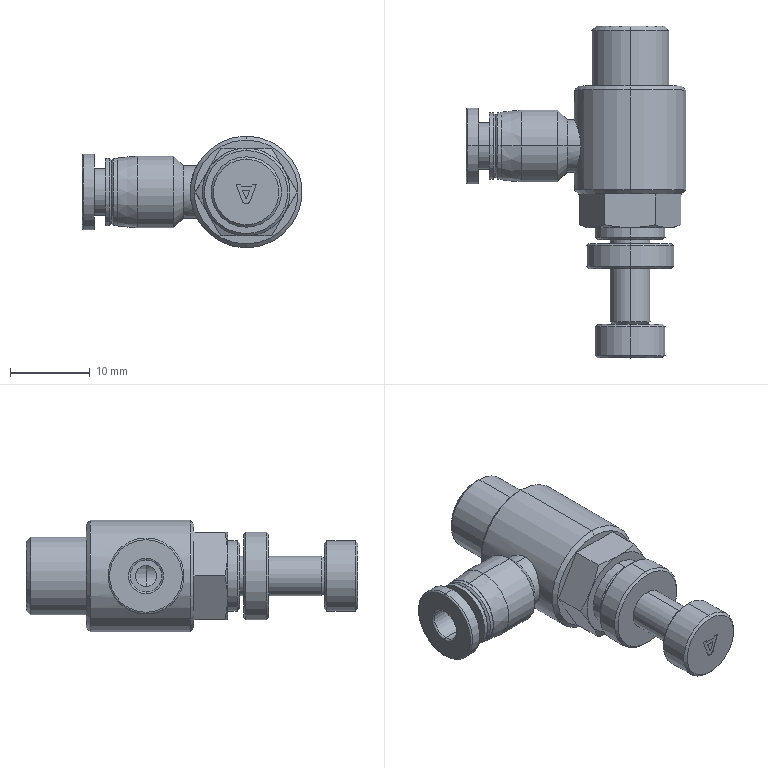Component | SolidWorks | F01AE00111-A2000-21TopEdgeAssembly-1_PSL401A-1 | 1 solid | 109 faces | box 27.5 x 41.5 x 14 mm | volume 4098 mm3 | cylinder 36 | plane 33 | cone 32 | torus 6 | sphere 2 | commonest cylinder face diameters 8.4 x4 8.8 x4 5 x4 2.667 x2 9 x2 5.8 x2 9.5 x2 6.6 x2
build123d program:
from build123d import *

# Parameters (mm, degrees)
SKETCH2_R          = 11
CUT_EXTRUDE1_DEPTH = 4.2
CUT_EXTRUDE2_DEPTH = 0.05


with BuildPart() as part:
    # Sketch1 → Revolve1 (revolve)
    with BuildSketch(Plane.XY, mode=Mode.PRIVATE) as revolve1_sk:
        Polygon((0, -15), (-4.283, -15), (-4.864, -14.419), (-4.864, -7.5), (-6.5, -7.5), (-7, -7), (-7, 5.5), (-6.5, 6), (-6.351, 6), (-6.351, 9.848), (-5.5, 10.2), (-4.4, 10.2), (-4.4, 11.4), (-4.1, 11.7), (-2.5, 11.7), (-2.5, 12.2), (-5.2, 12.2), (-5.5, 12.5), (-5.5, 15.05), (-5.2, 15.35), (-2.5, 15.35), (-2.5, 21.994), (-2.193, 22.3), (-4.1, 22.3), (-4.4, 22.6), (-4.4, 26.2), (-4.1, 26.5), (0, 26.5), align=None)
    revolve(revolve1_sk.sketch.rotate(Axis((0, 26.5, 0), (0, -1, 0)), 90), axis=Axis((0, 26.5, 0), (0, -1, 0)))

    # Sketch2 → Cut-Extrude1 (cut)
    with BuildSketch(Plane(origin=(0, 6, 0), x_dir=(1, 0, 0), z_dir=(0, 1, 0))):
        Circle(SKETCH2_R)
        Polygon((-6.351, 0), (-3.175, -5.5), (3.175, -5.5), (6.351, 0), (3.175, 5.5), (-3.175, 5.5), align=None, mode=Mode.SUBTRACT)
    extrude(amount=CUT_EXTRUDE1_DEPTH, mode=Mode.SUBTRACT)

    # Sketch3 → Revolve2 (revolve)
    with BuildSketch(Plane.XY, mode=Mode.PRIVATE) as revolve2_sk:
        with BuildLine():
            Line((0, 1.333), (6.5, 1.333))
            Line((6.5, 1.333), (6.5, 2))
            Line((6.5, 2), (20.3, 2))
            ThreePointArc((20.3, 2), (20.441, 2.059), (20.5, 2.2))
            Line((20.5, 2.2), (20.5, 4.55))
            ThreePointArc((20.5, 4.55), (20.441, 4.691), (20.3, 4.75))
            Line((20.3, 4.75), (19, 4.75))
            Line((19, 4.75), (19, 2.9))
            Line((19, 2.9), (17.6, 2.9))
            Line((17.6, 2.9), (17.6, 4.2))
            Line((17.6, 4.2), (17.1, 4.2))
            Line((17.1, 4.2), (16.85, 3.95))
            Line((16.85, 3.95), (16.6, 4.2))
            Line((16.6, 4.2), (16.1, 4.2))
            Line((16.1, 4.2), (16.1, 4.25))
            Line((16.1, 4.25), (13.6, 4.5))
            Line((13.6, 4.5), (9.071, 4.5))
            Line((9.071, 4.5), (7.871, 3.3))
            Line((7.871, 3.3), (0, 3.3))
            Line((0, 3.3), (0, 1.333))
        make_face()
    revolve(revolve2_sk.sketch.rotate(Axis((20.5, 0, 0), (-1, 0, 0)), 270), axis=Axis((20.5, 0, 0), (-1, 0, 0)))

    # Sketch4 → Cut-Revolve1 (revolve, cut)
    with BuildSketch(Plane.XY, mode=Mode.PRIVATE) as cut_revolve1_sk:
        with BuildLine():
            Line((0, -15), (-2.732, -15))
            ThreePointArc((-2.732, -15), (-2.52, -14.912), (-2.432, -14.7))
            Line((-2.432, -14.7), (-2.432, 0))
            Line((-2.432, 0), (-1.621, 0))
            Line((-1.621, 0), (-1.621, 1.621))
            ThreePointArc((-1.621, 1.621), (-1.146, 2.768), (0, 3.243))
            Line((0, 3.243), (0, -15))
        make_face()
    revolve(cut_revolve1_sk.sketch.rotate(Axis((0, 3.243, 0), (0, -1, 0)), 90), axis=Axis((0, 3.243, 0), (0, -1, 0)), mode=Mode.SUBTRACT)

    # Sketch5 → Cut-Revolve2 (revolve, cut)
    with BuildSketch(Plane.XY, mode=Mode.PRIVATE) as cut_revolve2_sk:
        Polygon((0, 0), (0, 1.333), (6.5, 1.333), (6.5, 2), (20.5, 2), (20.5, 0), align=None)
    revolve(cut_revolve2_sk.sketch.rotate(Axis((20.5, 0, 0), (-1, 0, 0)), 270), axis=Axis((20.5, 0, 0), (-1, 0, 0)), mode=Mode.SUBTRACT)

    # Sketch6 → Cut-Extrude2 (cut)
    with BuildSketch(Plane(origin=(0, 26.5, 0), x_dir=(1, 0, 0), z_dir=(0, 1, 0))):
        with BuildLine():
            Line((-1.26, -1), (-0.7279, -1))
            Line((-0.7279, -1), (-0.6369, -0.75))
            Line((-0.6369, -0.75), (0.6369, -0.75))
            Line((0.6369, -0.75), (0.7279, -1))
            Line((0.7279, -1), (1.26, -1))
            Line((1.26, -1), (0.4698, 1.171))
            ThreePointArc((0.4698, 1.171), (0, 1.5), (-0.4698, 1.171))
            Line((-0.4698, 1.171), (-1.26, -1))
        make_face()
        with BuildLine():
            Line((-0.455, -0.25), (0.455, -0.25))
            Line((0.455, -0.25), (0.09397, 0.7418))
            ThreePointArc((0.09397, 0.7418), (0, 0.8076), (-0.09397, 0.7418))
            Line((-0.09397, 0.7418), (-0.455, -0.25))
        make_face(mode=Mode.SUBTRACT)
    extrude(amount=-CUT_EXTRUDE2_DEPTH, mode=Mode.SUBTRACT)


solid = part.part

# Placed as in the assembly
solid = solid.moved(Location((-109.352, 62.048, -13.975), (0, 0, 180)))